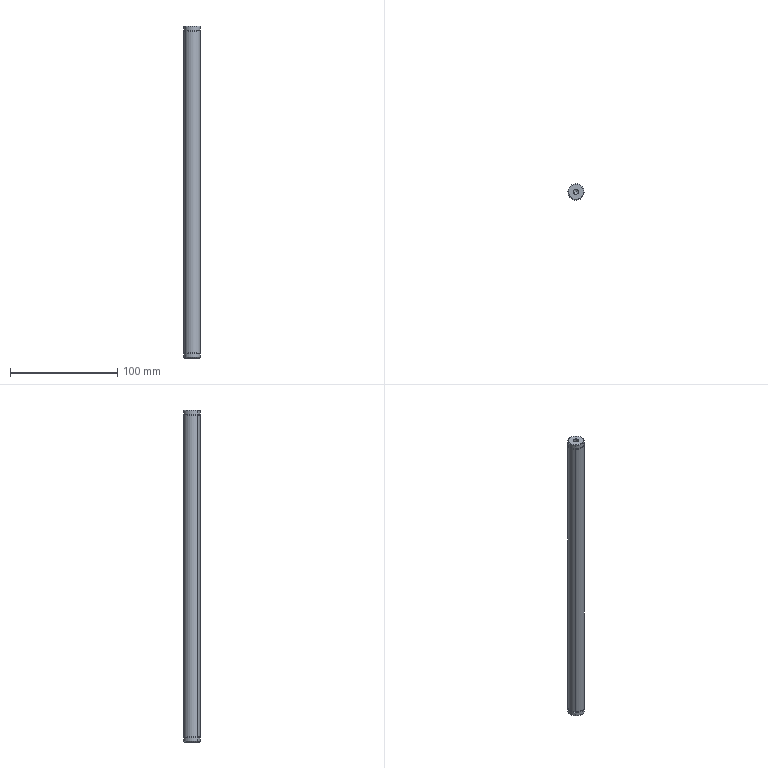Component | SolidWorks | KSD171005A-01-01-24-1 | 1 solid | 28 faces | box 15 x 15 x 310 mm | volume 54111 mm3 | cylinder 14 | cone 8 | plane 6 | commonest cylinder face diameters 15 x6 5 x4 14 x4 | material Chrome Plated Rod
build123d program:
from build123d import *

# Parameters (mm, degrees)
M6_TAPPED_HOLE3_D     = 5
M6_TAPPED_HOLE3_DEPTH = 15
M6_TAPPED_HOLE3_TIP   = 1.502
M6_TAPPED_HOLE2_D     = 5
M6_TAPPED_HOLE2_DEPTH = 15
M6_TAPPED_HOLE2_TIP   = 1.502
CHAMFER1_SIZE         = 0.5


with BuildPart() as part:
    # Sketch1 → Revolve1 (revolve)
    with BuildSketch(Plane.XY, mode=Mode.PRIVATE) as revolve1_sk:
        Polygon((0, 0), (0, 7.5), (3.9, 7.5), (3.9, 7), (5, 7), (5, 7.5), (305, 7.5), (305, 7), (306.1, 7), (306.1, 7.5), (310, 7.5), (310, 0), align=None)
    revolve(revolve1_sk.sketch.rotate(Axis((0, 0, 0), (1, 0, 0)), 90), axis=Axis((0, 0, 0), (1, 0, 0)))

    # M6 Tapped Hole3
    with Locations(Plane.ZY):
        with Locations((0, 0)):
            Hole(M6_TAPPED_HOLE3_D / 2, depth=M6_TAPPED_HOLE3_DEPTH)
            with Locations((0, 0, -(M6_TAPPED_HOLE3_DEPTH + M6_TAPPED_HOLE3_TIP / 2))):  # 118° drill point
                Cone(0, M6_TAPPED_HOLE3_D / 2, M6_TAPPED_HOLE3_TIP, mode=Mode.SUBTRACT)

    # M6 Tapped Hole2
    with Locations(Plane(origin=(310, 0, 0), x_dir=(0, 0, -1), z_dir=(1, 0, 0))):
        with Locations((0, 0)):
            Hole(M6_TAPPED_HOLE2_D / 2, depth=M6_TAPPED_HOLE2_DEPTH)
            with Locations((0, 0, -(M6_TAPPED_HOLE2_DEPTH + M6_TAPPED_HOLE2_TIP / 2))):  # 118° drill point
                Cone(0, M6_TAPPED_HOLE2_D / 2, M6_TAPPED_HOLE2_TIP, mode=Mode.SUBTRACT)

    # Chamfer1
    chamfer1_edges = [part.edges().sort_by_distance(p)[0] for p in [
        (0, 0, -7.5),
        (310, 0, -7.5),
    ]]
    chamfer(chamfer1_edges, length=CHAMFER1_SIZE)


solid = part.part

# Placed as in the assembly
solid = solid.moved(Location((-7.111, -209.27, 938), (0, 90, 0)))
STEP:
#1=COLOUR_RGB('',0.7922,0.8196,0.9333);
#2=FILL_AREA_STYLE_COLOUR('',#1);
#3=FILL_AREA_STYLE('',(#2));
#4=SURFACE_STYLE_FILL_AREA(#3);
#5=SURFACE_SIDE_STYLE('',(#4));
#6=SURFACE_STYLE_USAGE(.BOTH.,#5);
#7=PRESENTATION_STYLE_ASSIGNMENT((#6));
#8=CARTESIAN_POINT('',(-0.06473,-8.067,36.929));
#9=VERTEX_POINT('',#8);
#10=CARTESIAN_POINT('',(-0.4952,-8.411,36.929));
#11=VERTEX_POINT('',#10);
#12=CARTESIAN_POINT('',(-0.28,-8.239,36.929));
#13=DIRECTION('',(-0.,-0.,1.));
#14=DIRECTION('',(-0.781,-0.6245,0.));
#15=AXIS2_PLACEMENT_3D('',#12,#13,#14);
#16=CIRCLE('',#15,0.2756);
#17=EDGE_CURVE('',#9,#11,#16,.T.);
#18=ORIENTED_EDGE('',*,*,#17,.F.);
#19=CARTESIAN_POINT('',(-0.04936,-8.055,36.909));
#20=VERTEX_POINT('',#19);
#21=CARTESIAN_POINT('',(-0.04936,-8.055,36.909));
#22=DIRECTION('',(0.5523,0.4416,-0.7071));
#23=VECTOR('',#22,39.37);
#24=LINE('',#21,#23);
#25=EDGE_CURVE('',#9,#20,#24,.T.);
#26=ORIENTED_EDGE('',*,*,#25,.T.);
#27=CARTESIAN_POINT('',(-0.5106,-8.423,36.909));
#28=VERTEX_POINT('',#27);
#29=CARTESIAN_POINT('',(-0.28,-8.239,36.909));
#30=DIRECTION('',(0.,0.,-1.));
#31=DIRECTION('',(-0.781,-0.6245,0.));
#32=AXIS2_PLACEMENT_3D('',#29,#30,#31);
#33=CIRCLE('',#32,0.2953);
#34=EDGE_CURVE('',#28,#20,#33,.T.);
#35=ORIENTED_EDGE('',*,*,#34,.F.);
#36=CARTESIAN_POINT('',(-0.5106,-8.423,36.909));
#37=DIRECTION('',(-0.5523,-0.4416,-0.7071));
#38=VECTOR('',#37,39.37);
#39=LINE('',#36,#38);
#40=EDGE_CURVE('',#11,#28,#39,.T.);
#41=ORIENTED_EDGE('',*,*,#40,.F.);
#42=EDGE_LOOP('',(#18,#26,#35,#41));
#43=FACE_OUTER_BOUND('',#42,.T.);
#44=CARTESIAN_POINT('',(-0.28,-8.239,36.909));
#45=DIRECTION('',(0.,0.,-1.));
#46=DIRECTION('',(-0.781,-0.6245,0.));
#47=AXIS2_PLACEMENT_3D('',#44,#45,#46);
#48=CONICAL_SURFACE('',#47,0.2953,0.7854);
#49=ADVANCED_FACE('',(#43),#48,.T.);
#50=CARTESIAN_POINT('',(-0.4952,-8.411,24.724));
#51=VERTEX_POINT('',#50);
#52=CARTESIAN_POINT('',(-0.06473,-8.067,24.724));
#53=VERTEX_POINT('',#52);
#54=CARTESIAN_POINT('',(-0.28,-8.239,24.724));
#55=DIRECTION('',(0.,0.,-1.));
#56=DIRECTION('',(0.781,0.6245,0.));
#57=AXIS2_PLACEMENT_3D('',#54,#55,#56);
#58=CIRCLE('',#57,0.2756);
#59=EDGE_CURVE('',#51,#53,#58,.T.);
#60=ORIENTED_EDGE('',*,*,#59,.F.);
#61=CARTESIAN_POINT('',(-0.5106,-8.423,24.744));
#62=VERTEX_POINT('',#61);
#63=CARTESIAN_POINT('',(-0.4952,-8.411,24.724));
#64=DIRECTION('',(-0.5523,-0.4416,0.7071));
#65=VECTOR('',#64,39.37);
#66=LINE('',#63,#65);
#67=EDGE_CURVE('',#51,#62,#66,.T.);
#68=ORIENTED_EDGE('',*,*,#67,.T.);
#69=CARTESIAN_POINT('',(-0.04936,-8.055,24.744));
#70=VERTEX_POINT('',#69);
#71=CARTESIAN_POINT('',(-0.28,-8.239,24.744));
#72=DIRECTION('',(-0.,-0.,1.));
#73=DIRECTION('',(0.781,0.6245,0.));
#74=AXIS2_PLACEMENT_3D('',#71,#72,#73);
#75=CIRCLE('',#74,0.2953);
#76=EDGE_CURVE('',#70,#62,#75,.T.);
#77=ORIENTED_EDGE('',*,*,#76,.F.);
#78=CARTESIAN_POINT('',(-0.06473,-8.067,24.724));
#79=DIRECTION('',(0.5523,0.4416,0.7071));
#80=VECTOR('',#79,39.37);
#81=LINE('',#78,#80);
#82=EDGE_CURVE('',#53,#70,#81,.T.);
#83=ORIENTED_EDGE('',*,*,#82,.F.);
#84=EDGE_LOOP('',(#60,#68,#77,#83));
#85=FACE_OUTER_BOUND('',#84,.T.);
#86=CARTESIAN_POINT('',(-0.28,-8.239,24.724));
#87=DIRECTION('',(-0.,-0.,1.));
#88=DIRECTION('',(0.781,0.6245,0.));
#89=AXIS2_PLACEMENT_3D('',#86,#87,#88);
#90=CONICAL_SURFACE('',#89,0.2756,0.7854);
#91=ADVANCED_FACE('',(#85),#90,.T.);
#92=CARTESIAN_POINT('',(-0.3568,-8.3,36.339));
#93=VERTEX_POINT('',#92);
#94=CARTESIAN_POINT('',(-0.2031,-8.178,36.339));
#95=VERTEX_POINT('',#94);
#96=CARTESIAN_POINT('',(-0.28,-8.239,36.339));
#97=DIRECTION('',(-0.,-0.,1.));
#98=DIRECTION('',(0.781,0.6245,0.));
#99=AXIS2_PLACEMENT_3D('',#96,#97,#98);
#100=CIRCLE('',#99,0.09843);
#101=EDGE_CURVE('',#93,#95,#100,.T.);
#102=ORIENTED_EDGE('',*,*,#101,.F.);
#103=CARTESIAN_POINT('',(-0.3568,-8.3,36.929));
#104=VERTEX_POINT('',#103);
#105=CARTESIAN_POINT('',(-0.3568,-8.3,36.929));
#106=DIRECTION('',(-0.,-0.,1.));
#107=VECTOR('',#106,39.37);
#108=LINE('',#105,#107);
#109=EDGE_CURVE('',#93,#104,#108,.T.);
#110=ORIENTED_EDGE('',*,*,#109,.T.);
#111=CARTESIAN_POINT('',(-0.2031,-8.178,36.929));
#112=VERTEX_POINT('',#111);
#113=CARTESIAN_POINT('',(-0.28,-8.239,36.929));
#114=DIRECTION('',(-0.,-0.,1.));
#115=DIRECTION('',(0.781,0.6245,0.));
#116=AXIS2_PLACEMENT_3D('',#113,#114,#115);
#117=CIRCLE('',#116,0.09843);
#118=EDGE_CURVE('',#104,#112,#117,.T.);
#119=ORIENTED_EDGE('',*,*,#118,.T.);
#120=CARTESIAN_POINT('',(-0.2031,-8.178,36.929));
#121=DIRECTION('',(-0.,-0.,1.));
#122=VECTOR('',#121,39.37);
#123=LINE('',#120,#122);
#124=EDGE_CURVE('',#95,#112,#123,.T.);
#125=ORIENTED_EDGE('',*,*,#124,.F.);
#126=EDGE_LOOP('',(#102,#110,#119,#125));
#127=FACE_OUTER_BOUND('',#126,.T.);
#128=CARTESIAN_POINT('',(-0.28,-8.239,36.929));
#129=DIRECTION('',(-0.,-0.,1.));
#130=DIRECTION('',(0.781,0.6245,0.));
#131=AXIS2_PLACEMENT_3D('',#128,#129,#130);
#132=CYLINDRICAL_SURFACE('',#131,0.09843);
#133=ADVANCED_FACE('',(#127),#132,.F.);
#134=CARTESIAN_POINT('',(-0.28,-8.239,36.279));
#135=VERTEX_POINT('',#134);
#136=CARTESIAN_POINT('',(-0.2031,-8.178,36.339));
#137=DIRECTION('',(0.6695,0.5353,0.515));
#138=VECTOR('',#137,39.37);
#139=LINE('',#136,#138);
#140=EDGE_CURVE('',#135,#95,#139,.T.);
#141=ORIENTED_EDGE('',*,*,#140,.F.);
#142=CARTESIAN_POINT('',(-0.3568,-8.3,36.339));
#143=DIRECTION('',(-0.6695,-0.5353,0.515));
#144=VECTOR('',#143,39.37);
#145=LINE('',#142,#144);
#146=EDGE_CURVE('',#135,#93,#145,.T.);
#147=ORIENTED_EDGE('',*,*,#146,.T.);
#148=ORIENTED_EDGE('',*,*,#101,.T.);
#149=EDGE_LOOP('',(#141,#147,#148));
#150=FACE_OUTER_BOUND('',#149,.T.);
#151=CARTESIAN_POINT('',(-0.28,-8.239,36.339));
#152=DIRECTION('',(-0.,-0.,1.));
#153=DIRECTION('',(0.781,0.6245,0.));
#154=AXIS2_PLACEMENT_3D('',#151,#152,#153);
#155=CONICAL_SURFACE('',#154,0.09843,1.03);
#156=ADVANCED_FACE('',(#150),#155,.F.);
#157=CARTESIAN_POINT('',(-0.2031,-8.178,25.315));
#158=VERTEX_POINT('',#157);
#159=CARTESIAN_POINT('',(-0.3568,-8.3,25.315));
#160=VERTEX_POINT('',#159);
#161=CARTESIAN_POINT('',(-0.28,-8.239,25.315));
#162=DIRECTION('',(0.,0.,-1.));
#163=DIRECTION('',(-0.781,-0.6245,0.));
#164=AXIS2_PLACEMENT_3D('',#161,#162,#163);
#165=CIRCLE('',#164,0.09843);
#166=EDGE_CURVE('',#158,#160,#165,.T.);
#167=ORIENTED_EDGE('',*,*,#166,.F.);
#168=CARTESIAN_POINT('',(-0.2031,-8.178,24.724));
#169=VERTEX_POINT('',#168);
#170=CARTESIAN_POINT('',(-0.2031,-8.178,24.724));
#171=DIRECTION('',(0.,0.,-1.));
#172=VECTOR('',#171,39.37);
#173=LINE('',#170,#172);
#174=EDGE_CURVE('',#158,#169,#173,.T.);
#175=ORIENTED_EDGE('',*,*,#174,.T.);
#176=CARTESIAN_POINT('',(-0.3568,-8.3,24.724));
#177=VERTEX_POINT('',#176);
#178=CARTESIAN_POINT('',(-0.28,-8.239,24.724));
#179=DIRECTION('',(0.,0.,-1.));
#180=DIRECTION('',(-0.781,-0.6245,0.));
#181=AXIS2_PLACEMENT_3D('',#178,#179,#180);
#182=CIRCLE('',#181,0.09843);
#183=EDGE_CURVE('',#169,#177,#182,.T.);
#184=ORIENTED_EDGE('',*,*,#183,.T.);
#185=CARTESIAN_POINT('',(-0.3568,-8.3,24.724));
#186=DIRECTION('',(0.,0.,-1.));
#187=VECTOR('',#186,39.37);
#188=LINE('',#185,#187);
#189=EDGE_CURVE('',#160,#177,#188,.T.);
#190=ORIENTED_EDGE('',*,*,#189,.F.);
#191=EDGE_LOOP('',(#167,#175,#184,#190));
#192=FACE_OUTER_BOUND('',#191,.T.);
#193=CARTESIAN_POINT('',(-0.28,-8.239,24.724));
#194=DIRECTION('',(0.,0.,-1.));
#195=DIRECTION('',(-0.781,-0.6245,0.));
#196=AXIS2_PLACEMENT_3D('',#193,#194,#195);
#197=CYLINDRICAL_SURFACE('',#196,0.09843);
#198=ADVANCED_FACE('',(#192),#197,.F.);
#199=CARTESIAN_POINT('',(-0.28,-8.239,25.374));
#200=VERTEX_POINT('',#199);
#201=CARTESIAN_POINT('',(-0.3568,-8.3,25.315));
#202=DIRECTION('',(-0.6695,-0.5353,-0.515));
#203=VECTOR('',#202,39.37);
#204=LINE('',#201,#203);
#205=EDGE_CURVE('',#200,#160,#204,.T.);
#206=ORIENTED_EDGE('',*,*,#205,.F.);
#207=CARTESIAN_POINT('',(-0.2031,-8.178,25.315));
#208=DIRECTION('',(0.6695,0.5353,-0.515));
#209=VECTOR('',#208,39.37);
#210=LINE('',#207,#209);
#211=EDGE_CURVE('',#200,#158,#210,.T.);
#212=ORIENTED_EDGE('',*,*,#211,.T.);
#213=ORIENTED_EDGE('',*,*,#166,.T.);
#214=EDGE_LOOP('',(#206,#212,#213));
#215=FACE_OUTER_BOUND('',#214,.T.);
#216=CARTESIAN_POINT('',(-0.28,-8.239,25.315));
#217=DIRECTION('',(0.,0.,-1.));
#218=DIRECTION('',(-0.781,-0.6245,0.));
#219=AXIS2_PLACEMENT_3D('',#216,#217,#218);
#220=CONICAL_SURFACE('',#219,0.09843,1.03);
#221=ADVANCED_FACE('',(#215),#220,.F.);
#222=ORIENTED_EDGE('',*,*,#34,.T.);
#223=CARTESIAN_POINT('',(-0.04936,-8.055,36.776));
#224=VERTEX_POINT('',#223);
#225=CARTESIAN_POINT('',(-0.04936,-8.055,24.724));
#226=DIRECTION('',(0.,0.,-1.));
#227=VECTOR('',#226,39.37);
#228=LINE('',#225,#227);
#229=EDGE_CURVE('',#20,#224,#228,.T.);
#230=ORIENTED_EDGE('',*,*,#229,.T.);
#231=CARTESIAN_POINT('',(-0.5106,-8.423,36.776));
#232=VERTEX_POINT('',#231);
#233=CARTESIAN_POINT('',(-0.28,-8.239,36.776));
#234=DIRECTION('',(0.,0.,-1.));
#235=DIRECTION('',(-0.781,-0.6245,0.));
#236=AXIS2_PLACEMENT_3D('',#233,#234,#235);
#237=CIRCLE('',#236,0.2953);
#238=EDGE_CURVE('',#232,#224,#237,.T.);
#239=ORIENTED_EDGE('',*,*,#238,.F.);
#240=CARTESIAN_POINT('',(-0.5106,-8.423,24.724));
#241=DIRECTION('',(0.,0.,-1.));
#242=VECTOR('',#241,39.37);
#243=LINE('',#240,#242);
#244=EDGE_CURVE('',#28,#232,#243,.T.);
#245=ORIENTED_EDGE('',*,*,#244,.F.);
#246=EDGE_LOOP('',(#222,#230,#239,#245));
#247=FACE_OUTER_BOUND('',#246,.T.);
#248=CARTESIAN_POINT('',(-0.28,-8.239,24.724));
#249=DIRECTION('',(0.,0.,-1.));
#250=DIRECTION('',(-0.781,-0.6245,0.));
#251=AXIS2_PLACEMENT_3D('',#248,#249,#250);
#252=CYLINDRICAL_SURFACE('',#251,0.2953);
#253=ADVANCED_FACE('',(#247),#252,.T.);
#254=CARTESIAN_POINT('',(-0.4952,-8.411,36.776));
#255=VERTEX_POINT('',#254);
#256=CARTESIAN_POINT('',(-0.06473,-8.067,36.776));
#257=VERTEX_POINT('',#256);
#258=CARTESIAN_POINT('',(-0.28,-8.239,36.776));
#259=DIRECTION('',(0.,0.,-1.));
#260=DIRECTION('',(-0.781,-0.6245,0.));
#261=AXIS2_PLACEMENT_3D('',#258,#259,#260);
#262=CIRCLE('',#261,0.2756);
#263=EDGE_CURVE('',#255,#257,#262,.T.);
#264=ORIENTED_EDGE('',*,*,#263,.T.);
#265=CARTESIAN_POINT('',(-0.06473,-8.067,36.732));
#266=VERTEX_POINT('',#265);
#267=CARTESIAN_POINT('',(-0.06473,-8.067,24.724));
#268=DIRECTION('',(0.,0.,-1.));
#269=VECTOR('',#268,39.37);
#270=LINE('',#267,#269);
#271=EDGE_CURVE('',#257,#266,#270,.T.);
#272=ORIENTED_EDGE('',*,*,#271,.T.);
#273=CARTESIAN_POINT('',(-0.4952,-8.411,36.732));
#274=VERTEX_POINT('',#273);
#275=CARTESIAN_POINT('',(-0.28,-8.239,36.732));
#276=DIRECTION('',(0.,0.,-1.));
#277=DIRECTION('',(-0.781,-0.6245,0.));
#278=AXIS2_PLACEMENT_3D('',#275,#276,#277);
#279=CIRCLE('',#278,0.2756);
#280=EDGE_CURVE('',#274,#266,#279,.T.);
#281=ORIENTED_EDGE('',*,*,#280,.F.);
#282=CARTESIAN_POINT('',(-0.4952,-8.411,24.724));
#283=DIRECTION('',(0.,0.,-1.));
#284=VECTOR('',#283,39.37);
#285=LINE('',#282,#284);
#286=EDGE_CURVE('',#255,#274,#285,.T.);
#287=ORIENTED_EDGE('',*,*,#286,.F.);
#288=EDGE_LOOP('',(#264,#272,#281,#287));
#289=FACE_OUTER_BOUND('',#288,.T.);
#290=CARTESIAN_POINT('',(-0.28,-8.239,24.724));
#291=DIRECTION('',(0.,0.,-1.));
#292=DIRECTION('',(-0.781,-0.6245,0.));
#293=AXIS2_PLACEMENT_3D('',#290,#291,#292);
#294=CYLINDRICAL_SURFACE('',#293,0.2756);
#295=ADVANCED_FACE('',(#289),#294,.T.);
#296=CARTESIAN_POINT('',(-0.5106,-8.423,36.732));
#297=VERTEX_POINT('',#296);
#298=CARTESIAN_POINT('',(-0.04936,-8.055,36.732));
#299=VERTEX_POINT('',#298);
#300=CARTESIAN_POINT('',(-0.28,-8.239,36.732));
#301=DIRECTION('',(0.,0.,-1.));
#302=DIRECTION('',(-0.781,-0.6245,0.));
#303=AXIS2_PLACEMENT_3D('',#300,#301,#302);
#304=CIRCLE('',#303,0.2953);
#305=EDGE_CURVE('',#297,#299,#304,.T.);
#306=ORIENTED_EDGE('',*,*,#305,.T.);
#307=CARTESIAN_POINT('',(-0.04936,-8.055,24.921));
#308=VERTEX_POINT('',#307);
#309=CARTESIAN_POINT('',(-0.04936,-8.055,24.724));
#310=DIRECTION('',(0.,0.,-1.));
#311=VECTOR('',#310,39.37);
#312=LINE('',#309,#311);
#313=EDGE_CURVE('',#299,#308,#312,.T.);
#314=ORIENTED_EDGE('',*,*,#313,.T.);
#315=CARTESIAN_POINT('',(-0.5106,-8.423,24.921));
#316=VERTEX_POINT('',#315);
#317=CARTESIAN_POINT('',(-0.28,-8.239,24.921));
#318=DIRECTION('',(0.,0.,-1.));
#319=DIRECTION('',(-0.781,-0.6245,0.));
#320=AXIS2_PLACEMENT_3D('',#317,#318,#319);
#321=CIRCLE('',#320,0.2953);
#322=EDGE_CURVE('',#316,#308,#321,.T.);
#323=ORIENTED_EDGE('',*,*,#322,.F.);
#324=CARTESIAN_POINT('',(-0.5106,-8.423,24.724));
#325=DIRECTION('',(0.,0.,-1.));
#326=VECTOR('',#325,39.37);
#327=LINE('',#324,#326);
#328=EDGE_CURVE('',#297,#316,#327,.T.);
#329=ORIENTED_EDGE('',*,*,#328,.F.);
#330=EDGE_LOOP('',(#306,#314,#323,#329));
#331=FACE_OUTER_BOUND('',#330,.T.);
#332=CARTESIAN_POINT('',(-0.28,-8.239,24.724));
#333=DIRECTION('',(0.,0.,-1.));
#334=DIRECTION('',(-0.781,-0.6245,0.));
#335=AXIS2_PLACEMENT_3D('',#332,#333,#334);
#336=CYLINDRICAL_SURFACE('',#335,0.2953);
#337=ADVANCED_FACE('',(#331),#336,.T.);
#338=CARTESIAN_POINT('',(-0.4952,-8.411,24.921));
#339=VERTEX_POINT('',#338);
#340=CARTESIAN_POINT('',(-0.06473,-8.067,24.921));
#341=VERTEX_POINT('',#340);
#342=CARTESIAN_POINT('',(-0.28,-8.239,24.921));
#343=DIRECTION('',(0.,0.,-1.));
#344=DIRECTION('',(-0.781,-0.6245,0.));
#345=AXIS2_PLACEMENT_3D('',#342,#343,#344);
#346=CIRCLE('',#345,0.2756);
#347=EDGE_CURVE('',#339,#341,#346,.T.);
#348=ORIENTED_EDGE('',*,*,#347,.T.);
#349=CARTESIAN_POINT('',(-0.06473,-8.067,24.878));
#350=VERTEX_POINT('',#349);
#351=CARTESIAN_POINT('',(-0.06473,-8.067,24.724));
#352=DIRECTION('',(0.,0.,-1.));
#353=VECTOR('',#352,39.37);
#354=LINE('',#351,#353);
#355=EDGE_CURVE('',#341,#350,#354,.T.);
#356=ORIENTED_EDGE('',*,*,#355,.T.);
#357=CARTESIAN_POINT('',(-0.4952,-8.411,24.878));
#358=VERTEX_POINT('',#357);
#359=CARTESIAN_POINT('',(-0.28,-8.239,24.878));
#360=DIRECTION('',(0.,0.,-1.));
#361=DIRECTION('',(-0.781,-0.6245,0.));
#362=AXIS2_PLACEMENT_3D('',#359,#360,#361);
#363=CIRCLE('',#362,0.2756);
#364=EDGE_CURVE('',#358,#350,#363,.T.);
#365=ORIENTED_EDGE('',*,*,#364,.F.);
#366=CARTESIAN_POINT('',(-0.4952,-8.411,24.724));
#367=DIRECTION('',(0.,0.,-1.));
#368=VECTOR('',#367,39.37);
#369=LINE('',#366,#368);
#370=EDGE_CURVE('',#339,#358,#369,.T.);
#371=ORIENTED_EDGE('',*,*,#370,.F.);
#372=EDGE_LOOP('',(#348,#356,#365,#371));
#373=FACE_OUTER_BOUND('',#372,.T.);
#374=CARTESIAN_POINT('',(-0.28,-8.239,24.724));
#375=DIRECTION('',(0.,0.,-1.));
#376=DIRECTION('',(-0.781,-0.6245,0.));
#377=AXIS2_PLACEMENT_3D('',#374,#375,#376);
#378=CYLINDRICAL_SURFACE('',#377,0.2756);
#379=ADVANCED_FACE('',(#373),#378,.T.);
#380=CARTESIAN_POINT('',(-0.5106,-8.423,24.878));
#381=VERTEX_POINT('',#380);
#382=CARTESIAN_POINT('',(-0.04936,-8.055,24.878));
#383=VERTEX_POINT('',#382);
#384=CARTESIAN_POINT('',(-0.28,-8.239,24.878));
#385=DIRECTION('',(0.,0.,-1.));
#386=DIRECTION('',(-0.781,-0.6245,0.));
#387=AXIS2_PLACEMENT_3D('',#384,#385,#386);
#388=CIRCLE('',#387,0.2953);
#389=EDGE_CURVE('',#381,#383,#388,.T.);
#390=ORIENTED_EDGE('',*,*,#389,.T.);
#391=CARTESIAN_POINT('',(-0.04936,-8.055,24.724));
#392=DIRECTION('',(0.,0.,-1.));
#393=VECTOR('',#392,39.37);
#394=LINE('',#391,#393);
#395=EDGE_CURVE('',#383,#70,#394,.T.);
#396=ORIENTED_EDGE('',*,*,#395,.T.);
#397=ORIENTED_EDGE('',*,*,#76,.T.);
#398=CARTESIAN_POINT('',(-0.5106,-8.423,24.724));
#399=DIRECTION('',(0.,0.,-1.));
#400=VECTOR('',#399,39.37);
#401=LINE('',#398,#400);
#402=EDGE_CURVE('',#381,#62,#401,.T.);
#403=ORIENTED_EDGE('',*,*,#402,.F.);
#404=EDGE_LOOP('',(#390,#396,#397,#403));
#405=FACE_OUTER_BOUND('',#404,.T.);
#406=CARTESIAN_POINT('',(-0.28,-8.239,24.724));
#407=DIRECTION('',(0.,0.,-1.));
#408=DIRECTION('',(-0.781,-0.6245,0.));
#409=AXIS2_PLACEMENT_3D('',#406,#407,#408);
#410=CYLINDRICAL_SURFACE('',#409,0.2953);
#411=ADVANCED_FACE('',(#405),#410,.T.);
#412=CARTESIAN_POINT('',(-0.28,-8.239,24.724));
#413=DIRECTION('',(0.,0.,-1.));
#414=DIRECTION('',(0.781,0.6245,0.));
#415=AXIS2_PLACEMENT_3D('',#412,#413,#414);
#416=CIRCLE('',#415,0.2756);
#417=EDGE_CURVE('',#53,#51,#416,.T.);
#418=ORIENTED_EDGE('',*,*,#417,.T.);
#419=ORIENTED_EDGE('',*,*,#59,.T.);
#420=EDGE_LOOP('',(#418,#419));
#421=FACE_OUTER_BOUND('',#420,.T.);
#422=CARTESIAN_POINT('',(-0.28,-8.239,24.724));
#423=DIRECTION('',(0.,0.,-1.));
#424=DIRECTION('',(-0.781,-0.6245,0.));
#425=AXIS2_PLACEMENT_3D('',#422,#423,#424);
#426=CIRCLE('',#425,0.09843);
#427=EDGE_CURVE('',#177,#169,#426,.T.);
#428=ORIENTED_EDGE('',*,*,#427,.F.);
#429=ORIENTED_EDGE('',*,*,#183,.F.);
#430=EDGE_LOOP('',(#428,#429));
#431=FACE_BOUND('',#430,.T.);
#432=CARTESIAN_POINT('',(-0.28,-8.239,24.724));
#433=DIRECTION('',(0.,0.,1.));
#434=DIRECTION('',(0.781,0.6245,-0.));
#435=AXIS2_PLACEMENT_3D('',#432,#433,#434);
#436=PLANE('',#435);
#437=ADVANCED_FACE('',(#421,#431),#436,.F.);
#438=ORIENTED_EDGE('',*,*,#395,.F.);
#439=CARTESIAN_POINT('',(-0.28,-8.239,24.878));
#440=DIRECTION('',(0.,0.,-1.));
#441=DIRECTION('',(-0.781,-0.6245,0.));
#442=AXIS2_PLACEMENT_3D('',#439,#440,#441);
#443=CIRCLE('',#442,0.2953);
#444=EDGE_CURVE('',#383,#381,#443,.T.);
#445=ORIENTED_EDGE('',*,*,#444,.T.);
#446=ORIENTED_EDGE('',*,*,#402,.T.);
#447=CARTESIAN_POINT('',(-0.28,-8.239,24.744));
#448=DIRECTION('',(-0.,-0.,1.));
#449=DIRECTION('',(0.781,0.6245,0.));
#450=AXIS2_PLACEMENT_3D('',#447,#448,#449);
#451=CIRCLE('',#450,0.2953);
#452=EDGE_CURVE('',#62,#70,#451,.T.);
#453=ORIENTED_EDGE('',*,*,#452,.T.);
#454=EDGE_LOOP('',(#438,#445,#446,#453));
#455=FACE_OUTER_BOUND('',#454,.T.);
#456=CARTESIAN_POINT('',(-0.28,-8.239,24.724));
#457=DIRECTION('',(0.,0.,-1.));
#458=DIRECTION('',(-0.781,-0.6245,0.));
#459=AXIS2_PLACEMENT_3D('',#456,#457,#458);
#460=CYLINDRICAL_SURFACE('',#459,0.2953);
#461=ADVANCED_FACE('',(#455),#460,.T.);
#462=ORIENTED_EDGE('',*,*,#389,.F.);
#463=ORIENTED_EDGE('',*,*,#444,.F.);
#464=EDGE_LOOP('',(#462,#463));
#465=FACE_OUTER_BOUND('',#464,.T.);
#466=ORIENTED_EDGE('',*,*,#364,.T.);
#467=CARTESIAN_POINT('',(-0.28,-8.239,24.878));
#468=DIRECTION('',(0.,0.,-1.));
#469=DIRECTION('',(-0.781,-0.6245,0.));
#470=AXIS2_PLACEMENT_3D('',#467,#468,#469);
#471=CIRCLE('',#470,0.2756);
#472=EDGE_CURVE('',#350,#358,#471,.T.);
#473=ORIENTED_EDGE('',*,*,#472,.T.);
#474=EDGE_LOOP('',(#466,#473));
#475=FACE_BOUND('',#474,.T.);
#476=CARTESIAN_POINT('',(-0.4644,-8.008,24.878));
#477=DIRECTION('',(-0.,-0.,-1.));
#478=DIRECTION('',(-0.781,-0.6245,0.));
#479=AXIS2_PLACEMENT_3D('',#476,#477,#478);
#480=PLANE('',#479);
#481=ADVANCED_FACE('',(#465,#475),#480,.F.);
#482=ORIENTED_EDGE('',*,*,#355,.F.);
#483=CARTESIAN_POINT('',(-0.28,-8.239,24.921));
#484=DIRECTION('',(0.,0.,-1.));
#485=DIRECTION('',(-0.781,-0.6245,0.));
#486=AXIS2_PLACEMENT_3D('',#483,#484,#485);
#487=CIRCLE('',#486,0.2756);
#488=EDGE_CURVE('',#341,#339,#487,.T.);
#489=ORIENTED_EDGE('',*,*,#488,.T.);
#490=ORIENTED_EDGE('',*,*,#370,.T.);
#491=ORIENTED_EDGE('',*,*,#472,.F.);
#492=EDGE_LOOP('',(#482,#489,#490,#491));
#493=FACE_OUTER_BOUND('',#492,.T.);
#494=CARTESIAN_POINT('',(-0.28,-8.239,24.724));
#495=DIRECTION('',(0.,0.,-1.));
#496=DIRECTION('',(-0.781,-0.6245,0.));
#497=AXIS2_PLACEMENT_3D('',#494,#495,#496);
#498=CYLINDRICAL_SURFACE('',#497,0.2756);
#499=ADVANCED_FACE('',(#493),#498,.T.);
#500=ORIENTED_EDGE('',*,*,#347,.F.);
#501=ORIENTED_EDGE('',*,*,#488,.F.);
#502=EDGE_LOOP('',(#500,#501));
#503=FACE_BOUND('',#502,.T.);
#504=ORIENTED_EDGE('',*,*,#322,.T.);
#505=CARTESIAN_POINT('',(-0.28,-8.239,24.921));
#506=DIRECTION('',(0.,0.,-1.));
#507=DIRECTION('',(-0.781,-0.6245,0.));
#508=AXIS2_PLACEMENT_3D('',#505,#506,#507);
#509=CIRCLE('',#508,0.2953);
#510=EDGE_CURVE('',#308,#316,#509,.T.);
#511=ORIENTED_EDGE('',*,*,#510,.T.);
#512=EDGE_LOOP('',(#504,#511));
#513=FACE_OUTER_BOUND('',#512,.T.);
#514=CARTESIAN_POINT('',(-0.4521,-8.024,24.921));
#515=DIRECTION('',(0.,0.,1.));
#516=DIRECTION('',(0.781,0.6245,-0.));
#517=AXIS2_PLACEMENT_3D('',#514,#515,#516);
#518=PLANE('',#517);
#519=ADVANCED_FACE('',(#503,#513),#518,.F.);
#520=ORIENTED_EDGE('',*,*,#313,.F.);
#521=CARTESIAN_POINT('',(-0.28,-8.239,36.732));
#522=DIRECTION('',(0.,0.,-1.));
#523=DIRECTION('',(-0.781,-0.6245,0.));
#524=AXIS2_PLACEMENT_3D('',#521,#522,#523);
#525=CIRCLE('',#524,0.2953);
#526=EDGE_CURVE('',#299,#297,#525,.T.);
#527=ORIENTED_EDGE('',*,*,#526,.T.);
#528=ORIENTED_EDGE('',*,*,#328,.T.);
#529=ORIENTED_EDGE('',*,*,#510,.F.);
#530=EDGE_LOOP('',(#520,#527,#528,#529));
#531=FACE_OUTER_BOUND('',#530,.T.);
#532=CARTESIAN_POINT('',(-0.28,-8.239,24.724));
#533=DIRECTION('',(0.,0.,-1.));
#534=DIRECTION('',(-0.781,-0.6245,0.));
#535=AXIS2_PLACEMENT_3D('',#532,#533,#534);
#536=CYLINDRICAL_SURFACE('',#535,0.2953);
#537=ADVANCED_FACE('',(#531),#536,.T.);
#538=ORIENTED_EDGE('',*,*,#305,.F.);
#539=ORIENTED_EDGE('',*,*,#526,.F.);
#540=EDGE_LOOP('',(#538,#539));
#541=FACE_OUTER_BOUND('',#540,.T.);
#542=ORIENTED_EDGE('',*,*,#280,.T.);
#543=CARTESIAN_POINT('',(-0.28,-8.239,36.732));
#544=DIRECTION('',(0.,0.,-1.));
#545=DIRECTION('',(-0.781,-0.6245,0.));
#546=AXIS2_PLACEMENT_3D('',#543,#544,#545);
#547=CIRCLE('',#546,0.2756);
#548=EDGE_CURVE('',#266,#274,#547,.T.);
#549=ORIENTED_EDGE('',*,*,#548,.T.);
#550=EDGE_LOOP('',(#542,#549));
#551=FACE_BOUND('',#550,.T.);
#552=CARTESIAN_POINT('',(-0.4644,-8.008,36.732));
#553=DIRECTION('',(-0.,-0.,-1.));
#554=DIRECTION('',(-0.781,-0.6245,0.));
#555=AXIS2_PLACEMENT_3D('',#552,#553,#554);
#556=PLANE('',#555);
#557=ADVANCED_FACE('',(#541,#551),#556,.F.);
#558=ORIENTED_EDGE('',*,*,#271,.F.);
#559=CARTESIAN_POINT('',(-0.28,-8.239,36.776));
#560=DIRECTION('',(0.,0.,-1.));
#561=DIRECTION('',(-0.781,-0.6245,0.));
#562=AXIS2_PLACEMENT_3D('',#559,#560,#561);
#563=CIRCLE('',#562,0.2756);
#564=EDGE_CURVE('',#257,#255,#563,.T.);
#565=ORIENTED_EDGE('',*,*,#564,.T.);
#566=ORIENTED_EDGE('',*,*,#286,.T.);
#567=ORIENTED_EDGE('',*,*,#548,.F.);
#568=EDGE_LOOP('',(#558,#565,#566,#567));
#569=FACE_OUTER_BOUND('',#568,.T.);
#570=CARTESIAN_POINT('',(-0.28,-8.239,24.724));
#571=DIRECTION('',(0.,0.,-1.));
#572=DIRECTION('',(-0.781,-0.6245,0.));
#573=AXIS2_PLACEMENT_3D('',#570,#571,#572);
#574=CYLINDRICAL_SURFACE('',#573,0.2756);
#575=ADVANCED_FACE('',(#569),#574,.T.);
#576=ORIENTED_EDGE('',*,*,#263,.F.);
#577=ORIENTED_EDGE('',*,*,#564,.F.);
#578=EDGE_LOOP('',(#576,#577));
#579=FACE_BOUND('',#578,.T.);
#580=ORIENTED_EDGE('',*,*,#238,.T.);
#581=CARTESIAN_POINT('',(-0.28,-8.239,36.776));
#582=DIRECTION('',(0.,0.,-1.));
#583=DIRECTION('',(-0.781,-0.6245,0.));
#584=AXIS2_PLACEMENT_3D('',#581,#582,#583);
#585=CIRCLE('',#584,0.2953);
#586=EDGE_CURVE('',#224,#232,#585,.T.);
#587=ORIENTED_EDGE('',*,*,#586,.T.);
#588=EDGE_LOOP('',(#580,#587));
#589=FACE_OUTER_BOUND('',#588,.T.);
#590=CARTESIAN_POINT('',(-0.4521,-8.024,36.776));
#591=DIRECTION('',(0.,0.,1.));
#592=DIRECTION('',(0.781,0.6245,-0.));
#593=AXIS2_PLACEMENT_3D('',#590,#591,#592);
#594=PLANE('',#593);
#595=ADVANCED_FACE('',(#579,#589),#594,.F.);
#596=ORIENTED_EDGE('',*,*,#229,.F.);
#597=CARTESIAN_POINT('',(-0.28,-8.239,36.909));
#598=DIRECTION('',(0.,0.,-1.));
#599=DIRECTION('',(-0.781,-0.6245,0.));
#600=AXIS2_PLACEMENT_3D('',#597,#598,#599);
#601=CIRCLE('',#600,0.2953);
#602=EDGE_CURVE('',#20,#28,#601,.T.);
#603=ORIENTED_EDGE('',*,*,#602,.T.);
#604=ORIENTED_EDGE('',*,*,#244,.T.);
#605=ORIENTED_EDGE('',*,*,#586,.F.);
#606=EDGE_LOOP('',(#596,#603,#604,#605));
#607=FACE_OUTER_BOUND('',#606,.T.);
#608=CARTESIAN_POINT('',(-0.28,-8.239,24.724));
#609=DIRECTION('',(0.,0.,-1.));
#610=DIRECTION('',(-0.781,-0.6245,0.));
#611=AXIS2_PLACEMENT_3D('',#608,#609,#610);
#612=CYLINDRICAL_SURFACE('',#611,0.2953);
#613=ADVANCED_FACE('',(#607),#612,.T.);
#614=CARTESIAN_POINT('',(-0.28,-8.239,36.929));
#615=DIRECTION('',(-0.,-0.,1.));
#616=DIRECTION('',(-0.781,-0.6245,0.));
#617=AXIS2_PLACEMENT_3D('',#614,#615,#616);
#618=CIRCLE('',#617,0.2756);
#619=EDGE_CURVE('',#11,#9,#618,.T.);
#620=ORIENTED_EDGE('',*,*,#619,.T.);
#621=ORIENTED_EDGE('',*,*,#17,.T.);
#622=EDGE_LOOP('',(#620,#621));
#623=FACE_OUTER_BOUND('',#622,.T.);
#624=CARTESIAN_POINT('',(-0.28,-8.239,36.929));
#625=DIRECTION('',(-0.,-0.,1.));
#626=DIRECTION('',(0.781,0.6245,0.));
#627=AXIS2_PLACEMENT_3D('',#624,#625,#626);
#628=CIRCLE('',#627,0.09843);
#629=EDGE_CURVE('',#112,#104,#628,.T.);
#630=ORIENTED_EDGE('',*,*,#629,.F.);
#631=ORIENTED_EDGE('',*,*,#118,.F.);
#632=EDGE_LOOP('',(#630,#631));
#633=FACE_BOUND('',#632,.T.);
#634=CARTESIAN_POINT('',(-0.4644,-8.008,36.929));
#635=DIRECTION('',(-0.,-0.,-1.));
#636=DIRECTION('',(-0.781,-0.6245,0.));
#637=AXIS2_PLACEMENT_3D('',#634,#635,#636);
#638=PLANE('',#637);
#639=ADVANCED_FACE('',(#623,#633),#638,.F.);
#640=ORIENTED_EDGE('',*,*,#211,.F.);
#641=ORIENTED_EDGE('',*,*,#205,.T.);
#642=CARTESIAN_POINT('',(-0.28,-8.239,25.315));
#643=DIRECTION('',(0.,0.,-1.));
#644=DIRECTION('',(-0.781,-0.6245,0.));
#645=AXIS2_PLACEMENT_3D('',#642,#643,#644);
#646=CIRCLE('',#645,0.09843);
#647=EDGE_CURVE('',#160,#158,#646,.T.);
#648=ORIENTED_EDGE('',*,*,#647,.T.);
#649=EDGE_LOOP('',(#640,#641,#648));
#650=FACE_OUTER_BOUND('',#649,.T.);
#651=CARTESIAN_POINT('',(-0.28,-8.239,25.315));
#652=DIRECTION('',(0.,0.,-1.));
#653=DIRECTION('',(-0.781,-0.6245,0.));
#654=AXIS2_PLACEMENT_3D('',#651,#652,#653);
#655=CONICAL_SURFACE('',#654,0.09843,1.03);
#656=ADVANCED_FACE('',(#650),#655,.F.);
#657=ORIENTED_EDGE('',*,*,#174,.F.);
#658=ORIENTED_EDGE('',*,*,#647,.F.);
#659=ORIENTED_EDGE('',*,*,#189,.T.);
#660=ORIENTED_EDGE('',*,*,#427,.T.);
#661=EDGE_LOOP('',(#657,#658,#659,#660));
#662=FACE_OUTER_BOUND('',#661,.T.);
#663=CARTESIAN_POINT('',(-0.28,-8.239,24.724));
#664=DIRECTION('',(0.,0.,-1.));
#665=DIRECTION('',(-0.781,-0.6245,0.));
#666=AXIS2_PLACEMENT_3D('',#663,#664,#665);
#667=CYLINDRICAL_SURFACE('',#666,0.09843);
#668=ADVANCED_FACE('',(#662),#667,.F.);
#669=ORIENTED_EDGE('',*,*,#146,.F.);
#670=ORIENTED_EDGE('',*,*,#140,.T.);
#671=CARTESIAN_POINT('',(-0.28,-8.239,36.339));
#672=DIRECTION('',(-0.,-0.,1.));
#673=DIRECTION('',(0.781,0.6245,0.));
#674=AXIS2_PLACEMENT_3D('',#671,#672,#673);
#675=CIRCLE('',#674,0.09843);
#676=EDGE_CURVE('',#95,#93,#675,.T.);
#677=ORIENTED_EDGE('',*,*,#676,.T.);
#678=EDGE_LOOP('',(#669,#670,#677));
#679=FACE_OUTER_BOUND('',#678,.T.);
#680=CARTESIAN_POINT('',(-0.28,-8.239,36.339));
#681=DIRECTION('',(-0.,-0.,1.));
#682=DIRECTION('',(0.781,0.6245,0.));
#683=AXIS2_PLACEMENT_3D('',#680,#681,#682);
#684=CONICAL_SURFACE('',#683,0.09843,1.03);
#685=ADVANCED_FACE('',(#679),#684,.F.);
#686=ORIENTED_EDGE('',*,*,#109,.F.);
#687=ORIENTED_EDGE('',*,*,#676,.F.);
#688=ORIENTED_EDGE('',*,*,#124,.T.);
#689=ORIENTED_EDGE('',*,*,#629,.T.);
#690=EDGE_LOOP('',(#686,#687,#688,#689));
#691=FACE_OUTER_BOUND('',#690,.T.);
#692=CARTESIAN_POINT('',(-0.28,-8.239,36.929));
#693=DIRECTION('',(-0.,-0.,1.));
#694=DIRECTION('',(0.781,0.6245,0.));
#695=AXIS2_PLACEMENT_3D('',#692,#693,#694);
#696=CYLINDRICAL_SURFACE('',#695,0.09843);
#697=ADVANCED_FACE('',(#691),#696,.F.);
#698=ORIENTED_EDGE('',*,*,#67,.F.);
#699=ORIENTED_EDGE('',*,*,#417,.F.);
#700=ORIENTED_EDGE('',*,*,#82,.T.);
#701=ORIENTED_EDGE('',*,*,#452,.F.);
#702=EDGE_LOOP('',(#698,#699,#700,#701));
#703=FACE_OUTER_BOUND('',#702,.T.);
#704=CARTESIAN_POINT('',(-0.28,-8.239,24.724));
#705=DIRECTION('',(-0.,-0.,1.));
#706=DIRECTION('',(0.781,0.6245,0.));
#707=AXIS2_PLACEMENT_3D('',#704,#705,#706);
#708=CONICAL_SURFACE('',#707,0.2756,0.7854);
#709=ADVANCED_FACE('',(#703),#708,.T.);
#710=ORIENTED_EDGE('',*,*,#25,.F.);
#711=ORIENTED_EDGE('',*,*,#619,.F.);
#712=ORIENTED_EDGE('',*,*,#40,.T.);
#713=ORIENTED_EDGE('',*,*,#602,.F.);
#714=EDGE_LOOP('',(#710,#711,#712,#713));
#715=FACE_OUTER_BOUND('',#714,.T.);
#716=CARTESIAN_POINT('',(-0.28,-8.239,36.909));
#717=DIRECTION('',(0.,0.,-1.));
#718=DIRECTION('',(-0.781,-0.6245,0.));
#719=AXIS2_PLACEMENT_3D('',#716,#717,#718);
#720=CONICAL_SURFACE('',#719,0.2953,0.7854);
#721=ADVANCED_FACE('',(#715),#720,.T.);
#722=CLOSED_SHELL('',(#49,#91,#133,#156,#198,#221,#253,#295,#337,#379,#411,#437,#461,#481,#499,#519,#537,#557,#575,#595,#613,#639,#656,#668,#685,#697,#709,#721));
#723=MANIFOLD_SOLID_BREP('',#722);
#724=STYLED_ITEM('',(#7),#723);
#725=(LENGTH_UNIT()NAMED_UNIT(*)SI_UNIT($,.METRE.));
#726=LENGTH_MEASURE_WITH_UNIT(LENGTH_MEASURE(0.0254),#725);
#727=DIMENSIONAL_EXPONENTS(1.,0.,0.,0.,0.,0.,0.);
#728=(CONVERSION_BASED_UNIT('',#726)LENGTH_UNIT()NAMED_UNIT(#727));
#729=UNCERTAINTY_MEASURE_WITH_UNIT(LENGTH_MEASURE(0.00001),#728,'','');
#730=(NAMED_UNIT(*)PLANE_ANGLE_UNIT()SI_UNIT($,.RADIAN.));
#731=(NAMED_UNIT(*)SI_UNIT($,.STERADIAN.)SOLID_ANGLE_UNIT());
#732=(GEOMETRIC_REPRESENTATION_CONTEXT(3)GLOBAL_UNCERTAINTY_ASSIGNED_CONTEXT((#729))GLOBAL_UNIT_ASSIGNED_CONTEXT((#728,#730,#731))REPRESENTATION_CONTEXT('',''));
#733=MECHANICAL_DESIGN_GEOMETRIC_PRESENTATION_REPRESENTATION('',(#724),#732);
#734=CARTESIAN_POINT('',(0.,0.,0.));
#735=DIRECTION('',(0.,0.,1.));
#736=DIRECTION('',(1.,0.,0.));
#737=AXIS2_PLACEMENT_3D('',#734,#735,#736);
#738=(LENGTH_UNIT()NAMED_UNIT(*)SI_UNIT($,.METRE.));
#739=LENGTH_MEASURE_WITH_UNIT(LENGTH_MEASURE(0.0254),#738);
#740=DIMENSIONAL_EXPONENTS(1.,0.,0.,0.,0.,0.,0.);
#741=(CONVERSION_BASED_UNIT('',#739)LENGTH_UNIT()NAMED_UNIT(#740));
#742=UNCERTAINTY_MEASURE_WITH_UNIT(LENGTH_MEASURE(0.00001),#741,'','');
#743=(NAMED_UNIT(*)PLANE_ANGLE_UNIT()SI_UNIT($,.RADIAN.));
#744=(NAMED_UNIT(*)SI_UNIT($,.STERADIAN.)SOLID_ANGLE_UNIT());
#745=(GEOMETRIC_REPRESENTATION_CONTEXT(3)GLOBAL_UNCERTAINTY_ASSIGNED_CONTEXT((#742))GLOBAL_UNIT_ASSIGNED_CONTEXT((#741,#743,#744))REPRESENTATION_CONTEXT('',''));
#746=ADVANCED_BREP_SHAPE_REPRESENTATION('',(#723,#737),#745);
#747=PRESENTATION_LAYER_ASSIGNMENT('','',(#724));